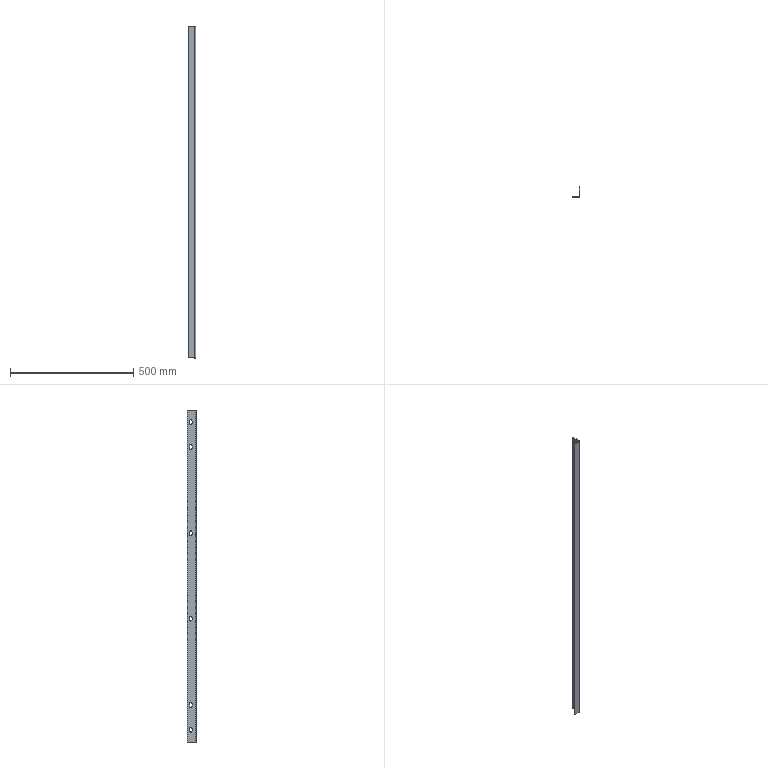Component | SolidWorks | FrontSidePlateAssembly-1_FrontSidePanelReinforcementVerticalRib-1 | 1 solid | 46 faces | volume 177118 mm3 | plane 26 | cylinder 20 | commonest cylinder face diameters 10 x18 8 x1 4 x1 | material Plain Carbon Steel